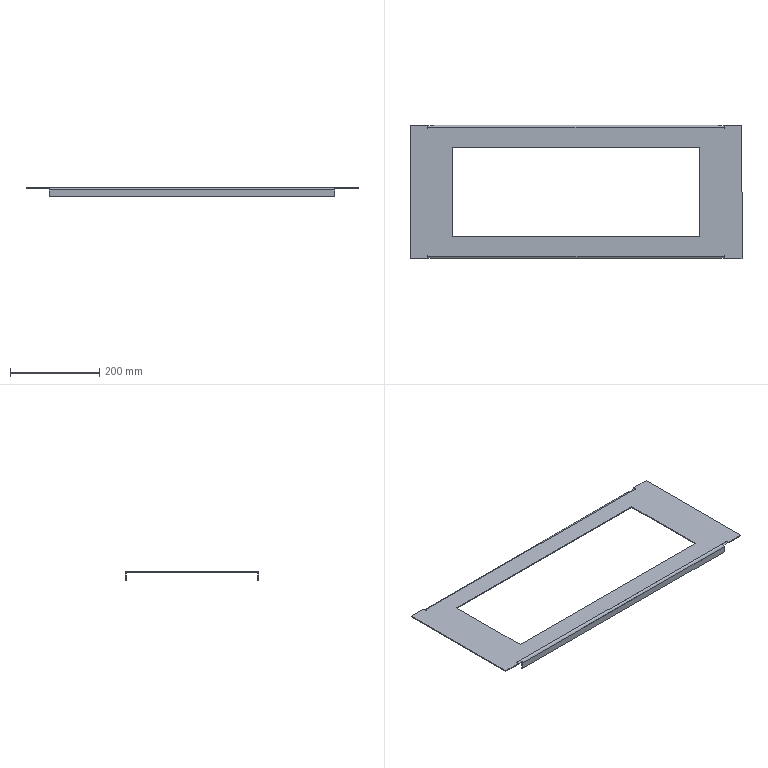Component | SolidWorks | Panel3-2 | 1 solid | 42 faces | volume 264317 mm3 | plane 38 | cylinder 4 | commonest cylinder face diameters 11 x2 7 x2 | material Malleable Cast Iron